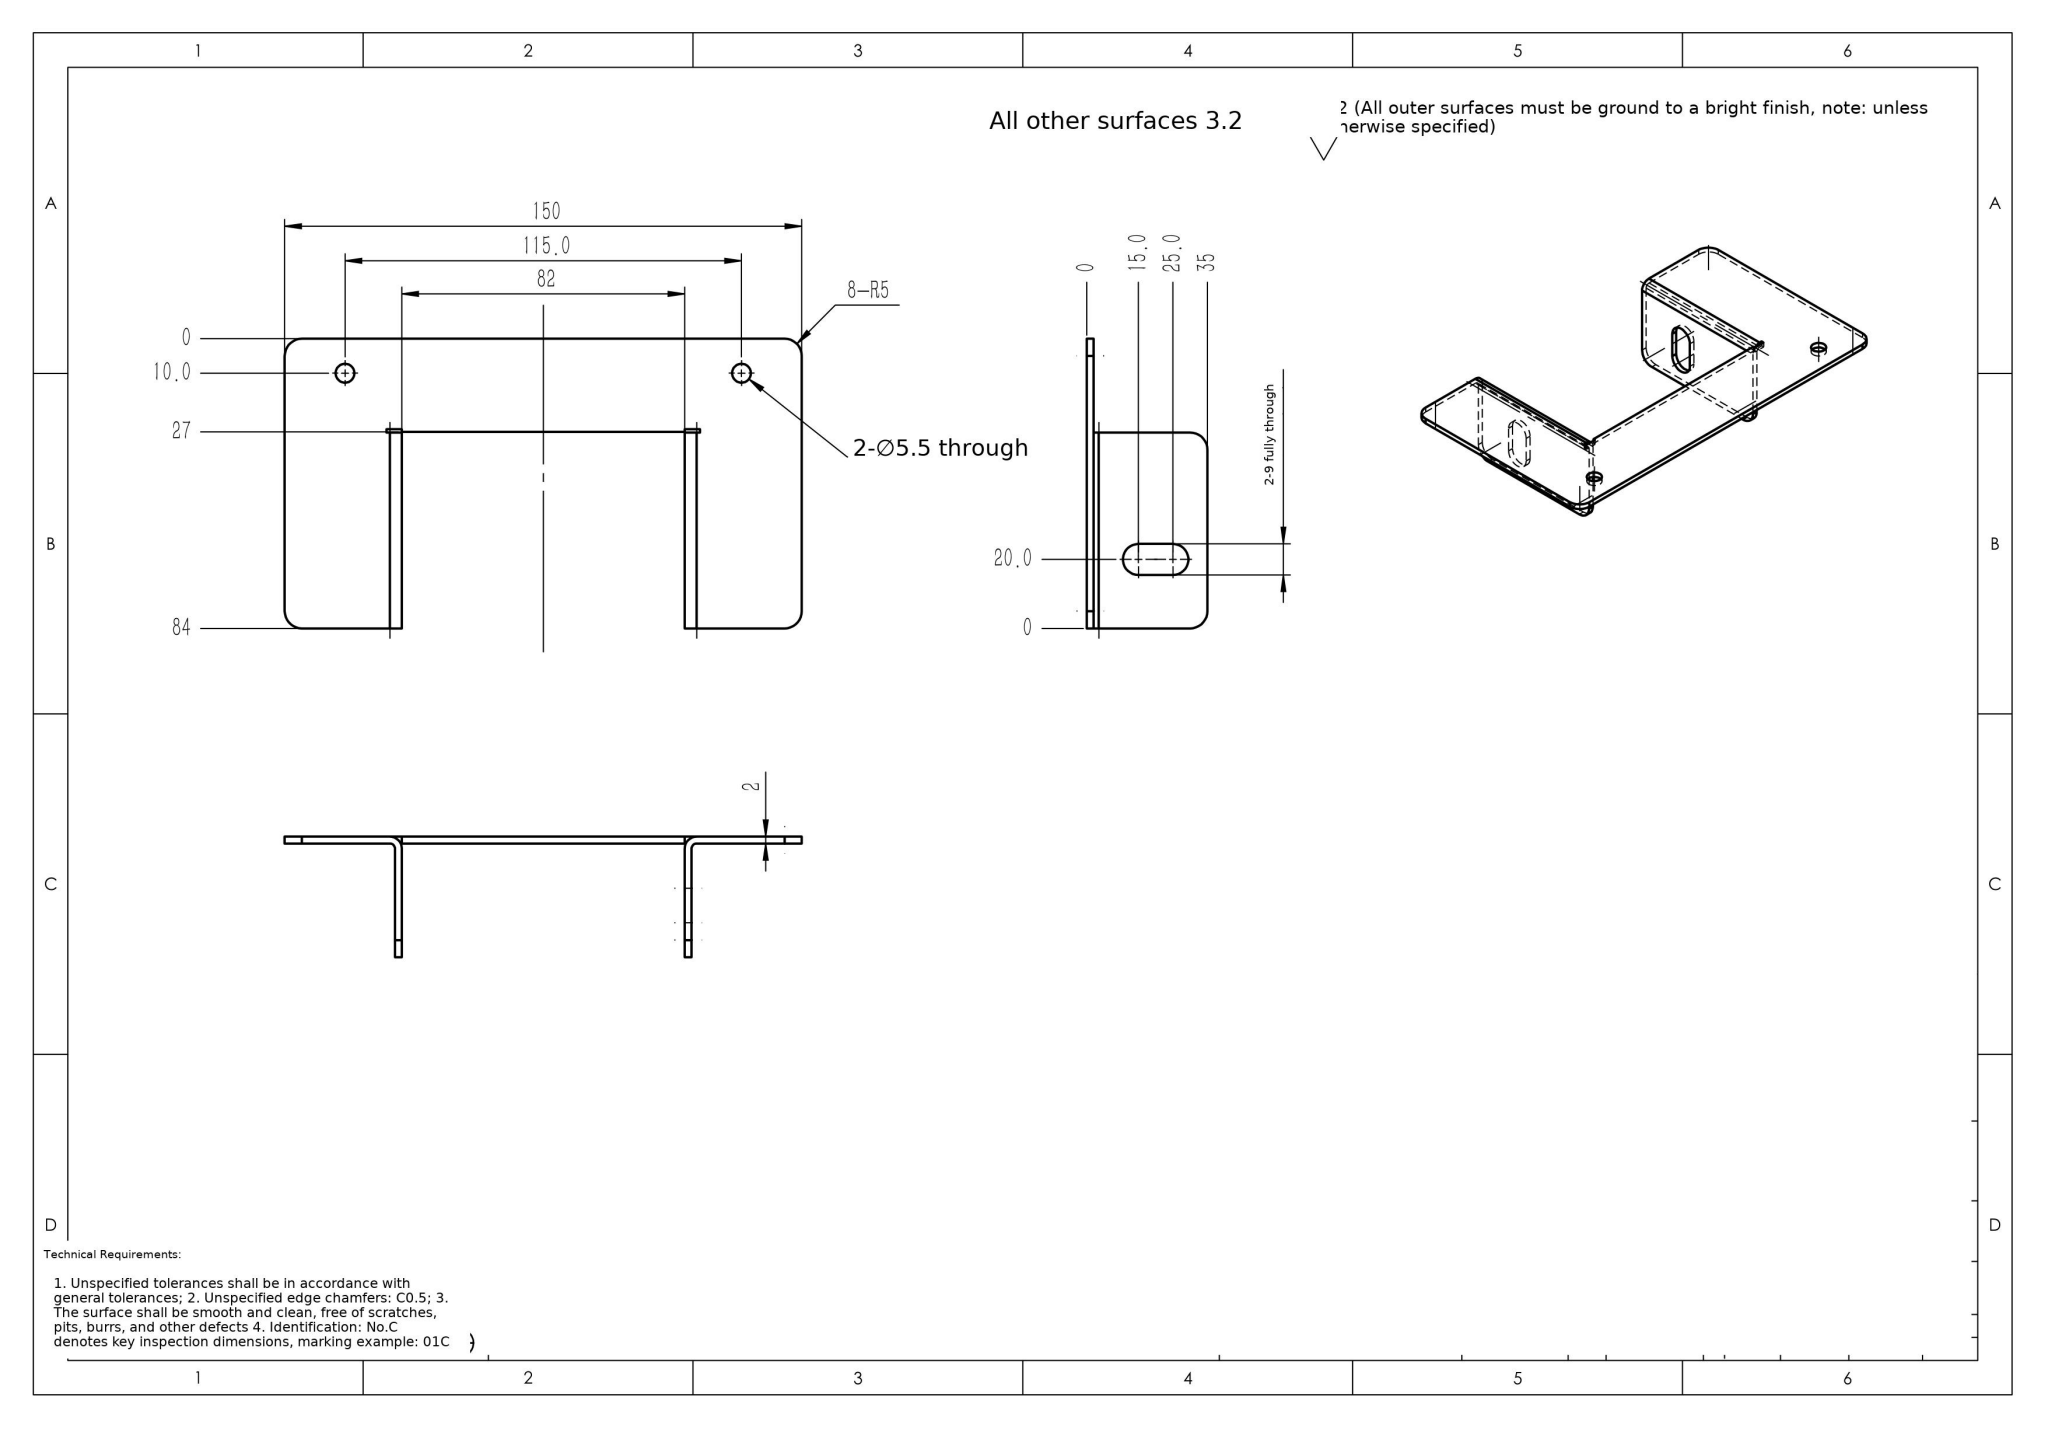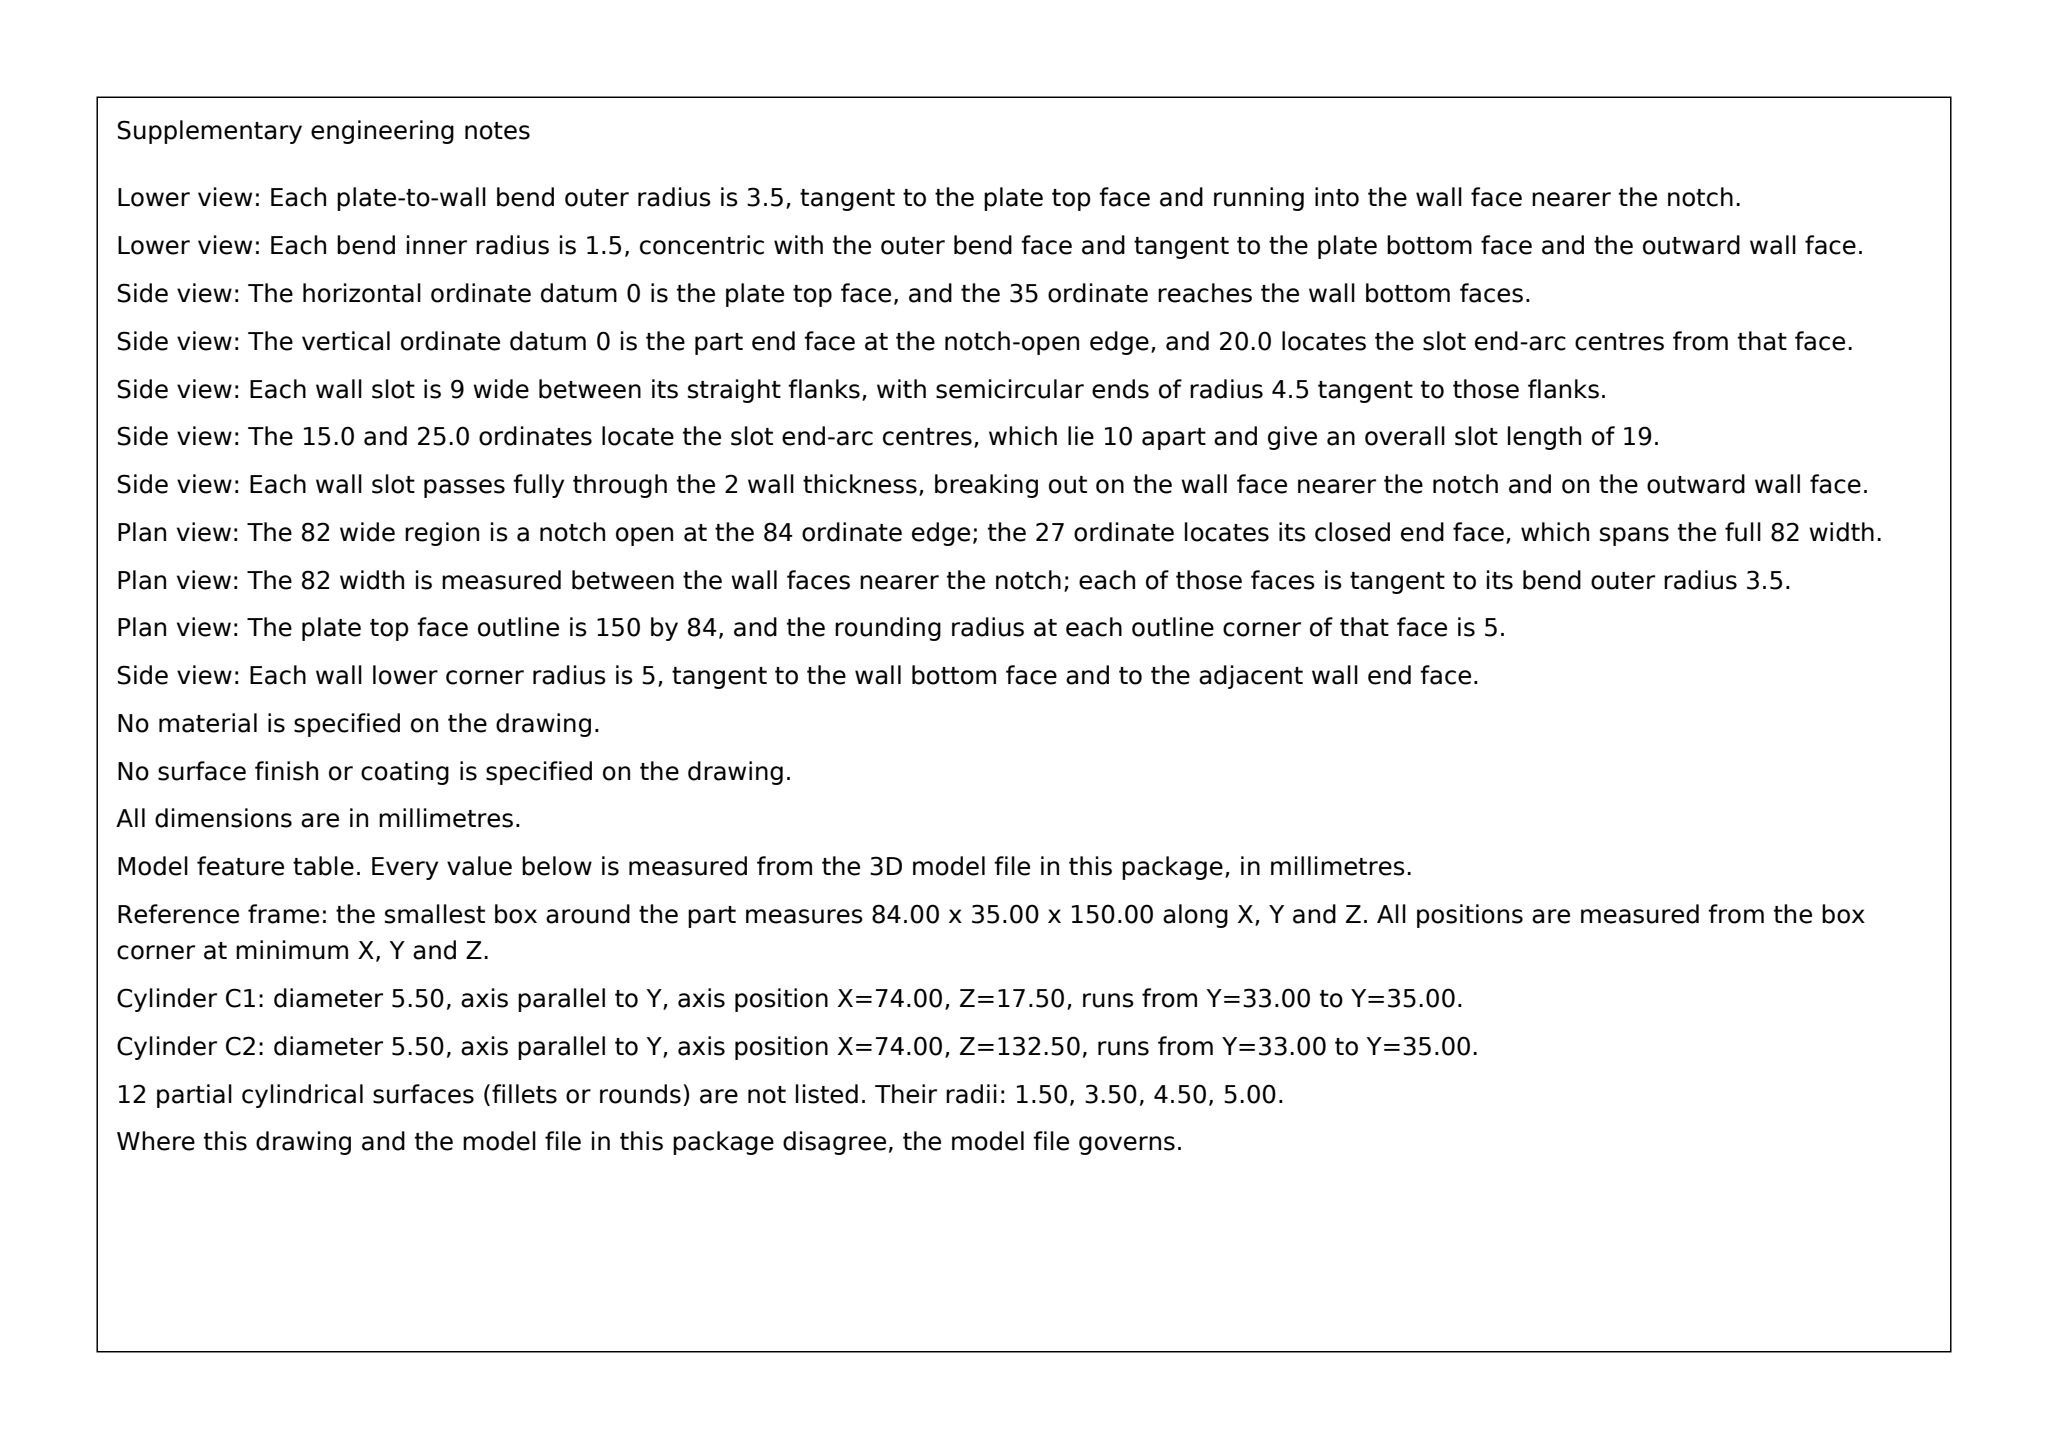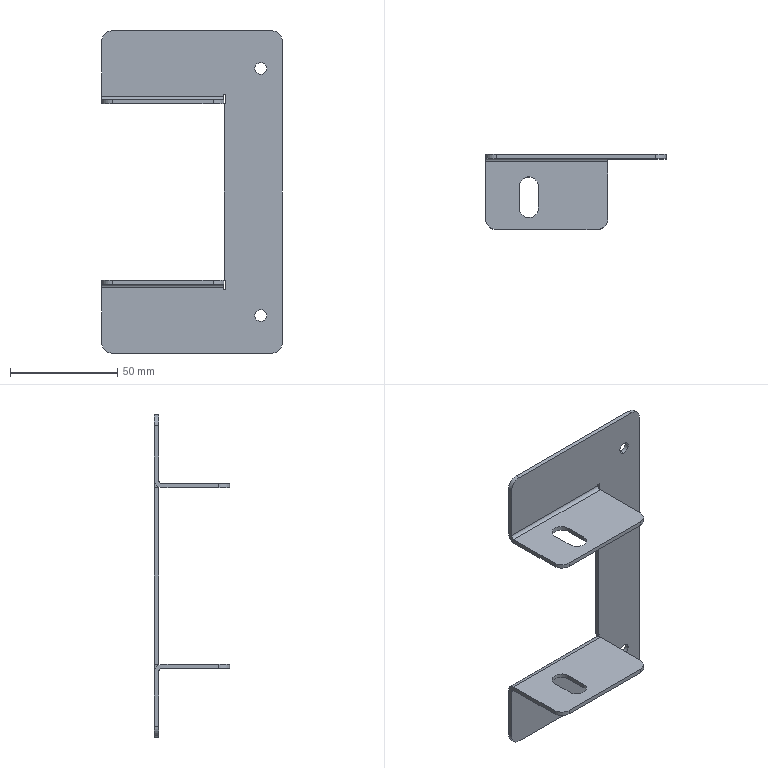Part | SolidWorks | mm | 1 solid | 46 faces | box 84 x 35 x 150 mm | volume 22292 mm3 | plane 26 | cylinder 20 | commonest cylinder face diameters 10 x8 5.5 x4 9 x4 3 x2 7 x2
Drawing notes:
SLOT 2X Ø9 THRU (OBROUND 9 WIDE X 19 LONG), END CENTRES 10.0 AND 20.0 FROM BOTTOM EDGE, 20.0 FROM BACK FACE; TYP. BOTH UPRIGHT FLANGES | from the solid: cylinders [9.0,"z",[20.0,10.0,null],2.0,2] and [9.0,"z",[20.0,20.0,null],2.0,2]
ALL DIMENSIONS IN MILLIMETERS | from the solid: STEP model facts header: units mm; bbox_xyz [84.0, 35.0, 150.0]
MATERIAL THICKNESS 2 THRU (FLANGE WALL): FACES AT Z=0/2 AND Z=118/120.5 REF, PLATE FACES Y=33/35 | from the solid: axis_planes ["z",0.0],["z",118.0],["z",120.5],["y",33.0],["y",35.0]
2X Ø9 THRU (slot ends), slot centreline 20 from side-flange front face, hole centres 10 and 20 from bottom face | from the solid: cylinders [9.0,"z",[20.0,10.0],2.0] and [9.0,"z",[20.0,20.0],2.0]
ALL DIMENSIONS IN MILLIMETRES | from the solid: STEP model facts stated in mm, bbox_xyz [84.0, 35.0, 150.0]
SLOT 9 WIDE x 19 LONG THRU 2 THK FLANGE (2X R4.5 ENDS), SLOT AXIS NORMAL TO FLANGE; END CENTERS AT X=20, Y=10 AND Y=20 FROM BBOX MIN CORNER | from the solid: cylinders [9.0,'z',[20.0,10.0],2.0] and [9.0,'z',[20.0,20.0],2.0]; x-planes 15.5 and 24.5; plate thickness from y/z 2.0 wall